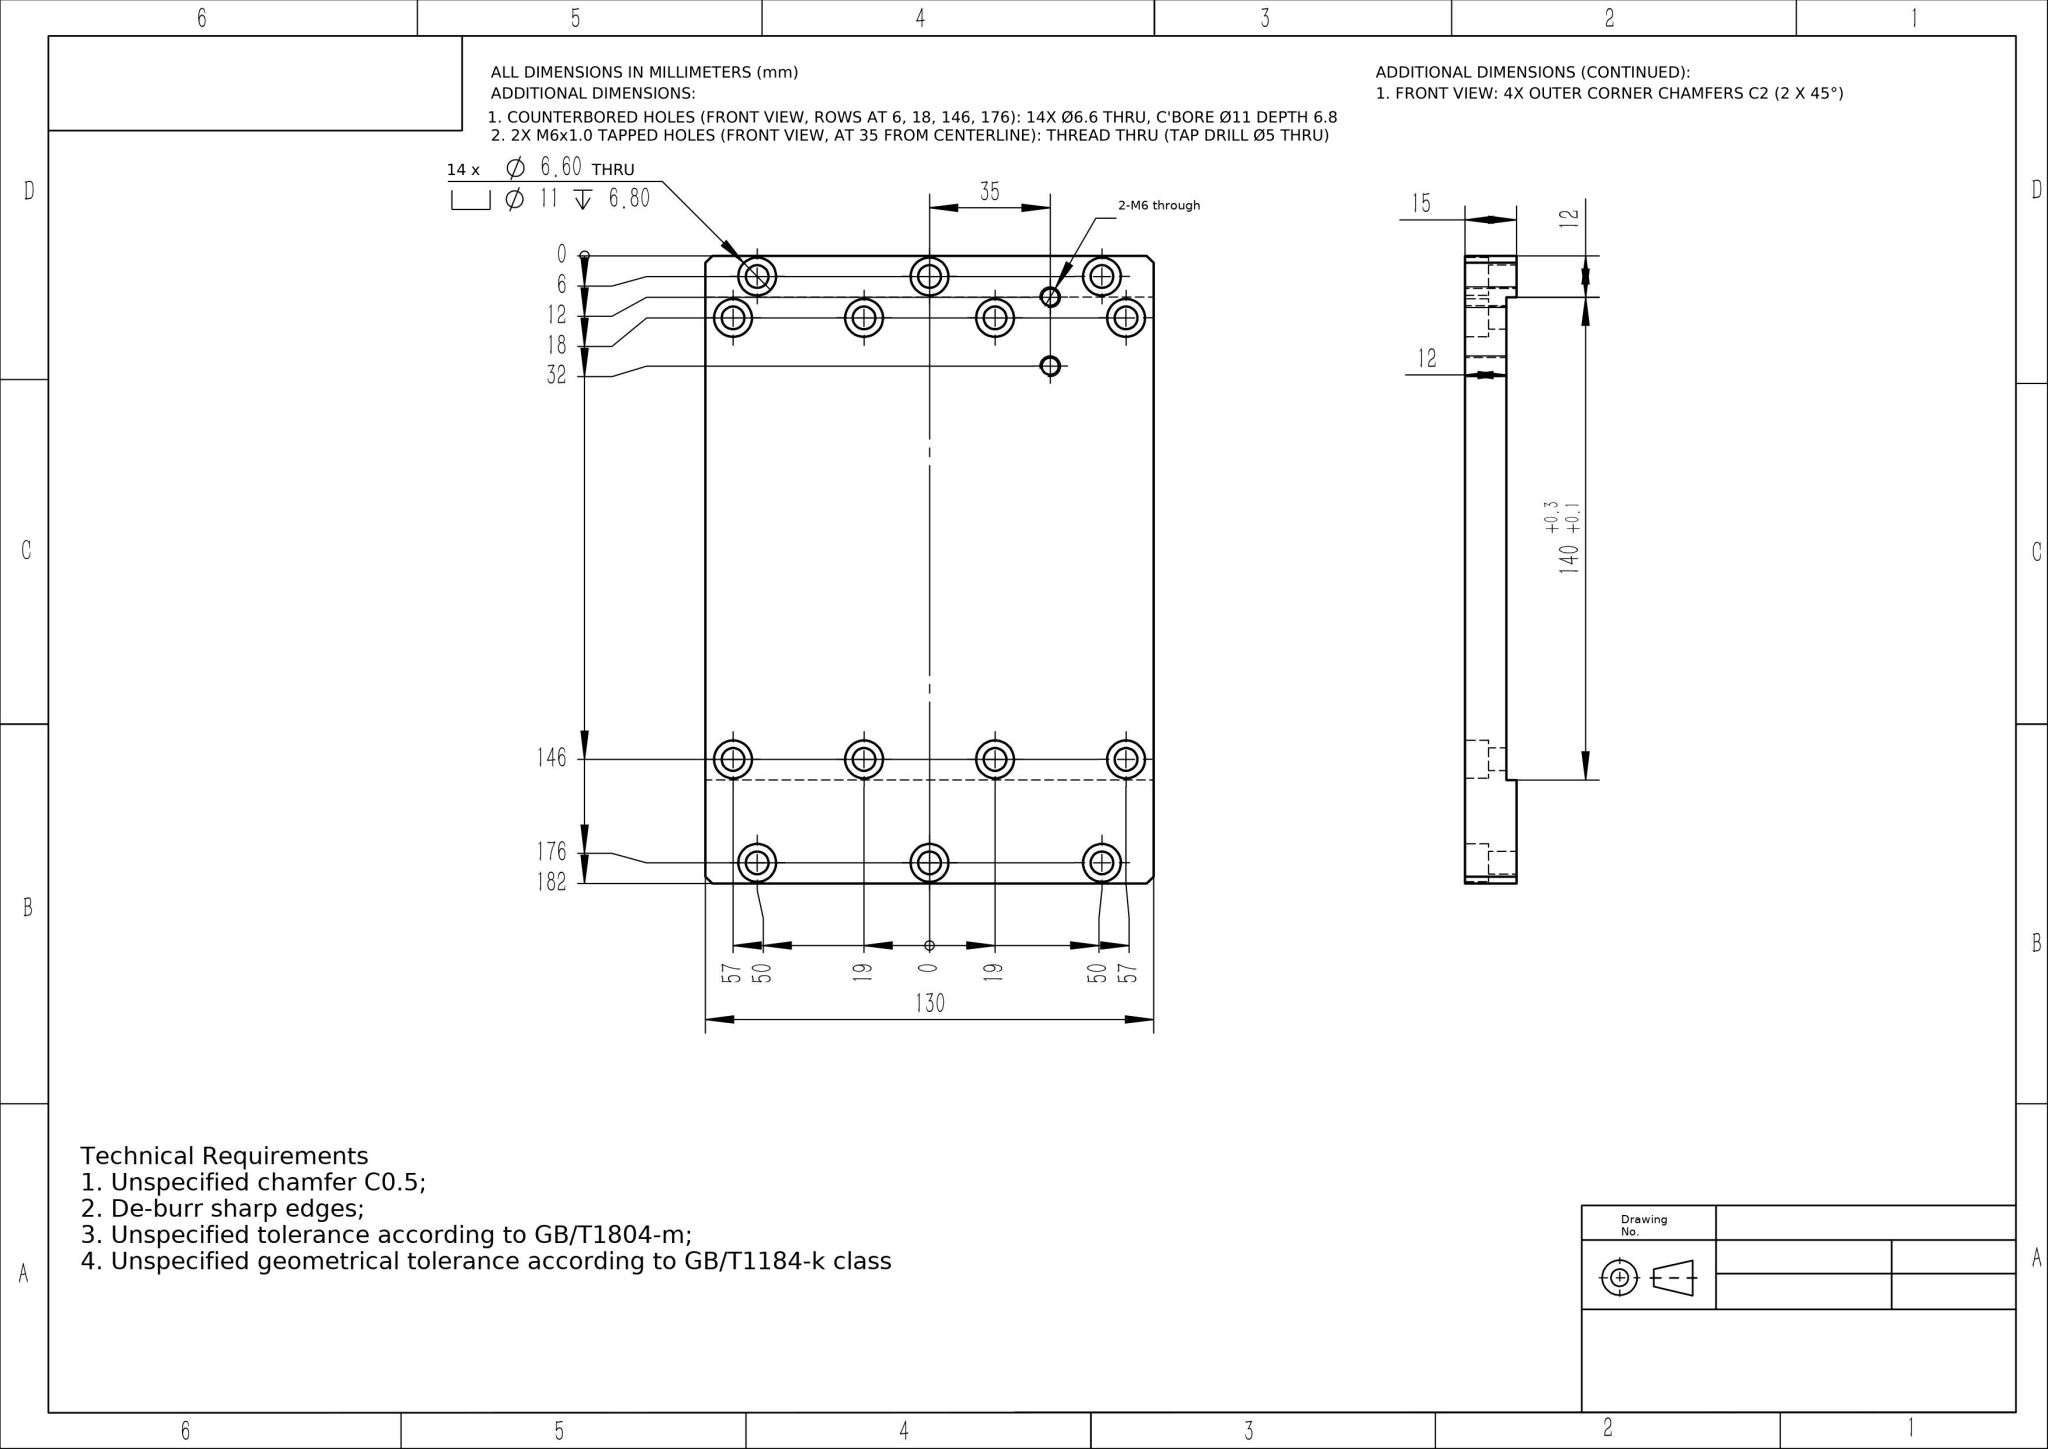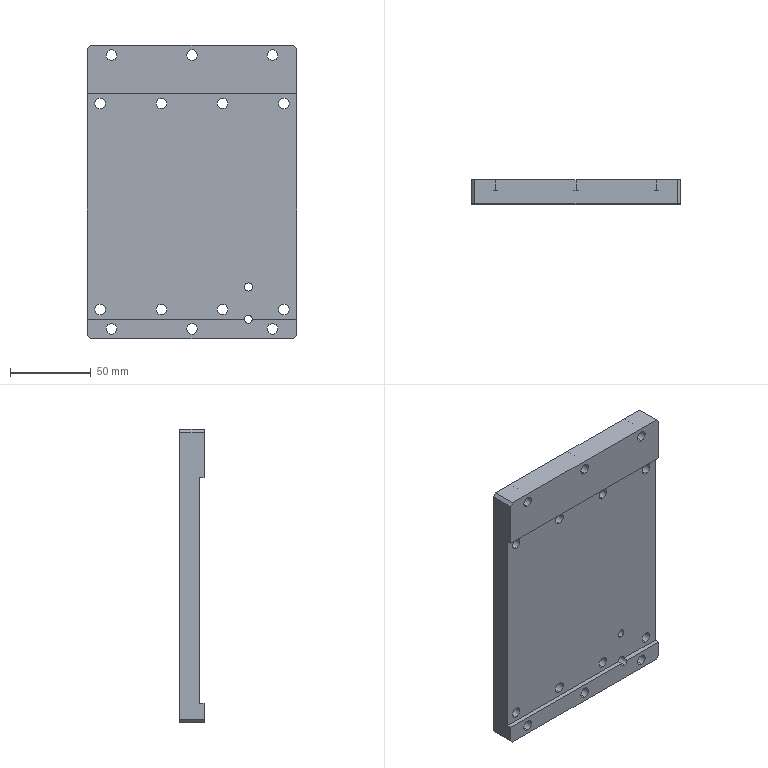Part | NX | mm | 1 solid | 89 faces | box 130 x 15 x 182 mm | volume 287526 mm3 | cylinder 60 | plane 29 | commonest cylinder face diameters 11 x28 6.6 x28 5 x4